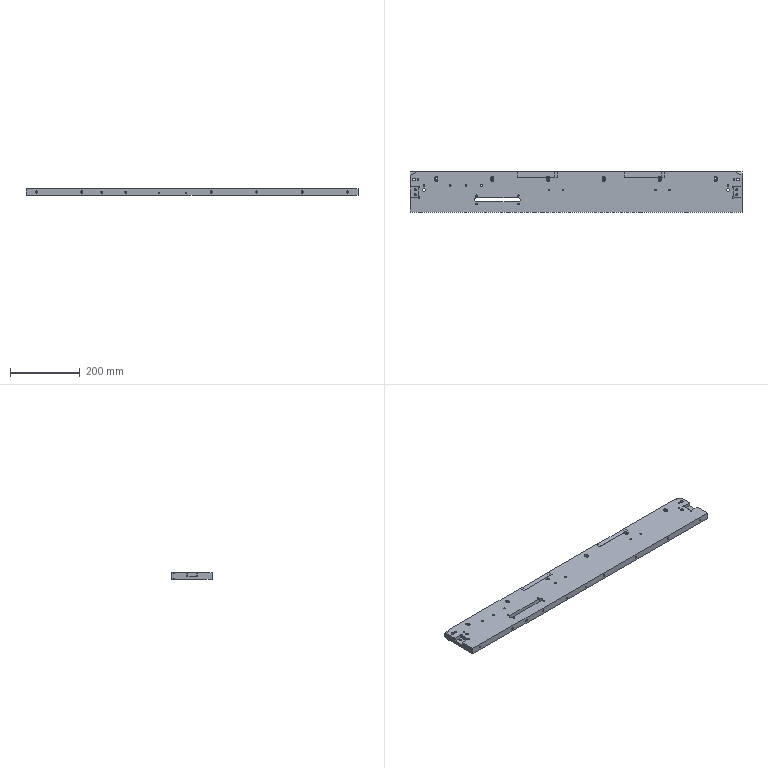Component | SolidWorks | --MA18S20041SidePlate2-1 | 1 solid | 203 faces | volume 2009269 mm3 | cylinder 119 | plane 64 | cone 20 | commonest cylinder face diameters 5 x56 4.2 x20 6 x16 10 x12 8 x8 50 x4 11 x3